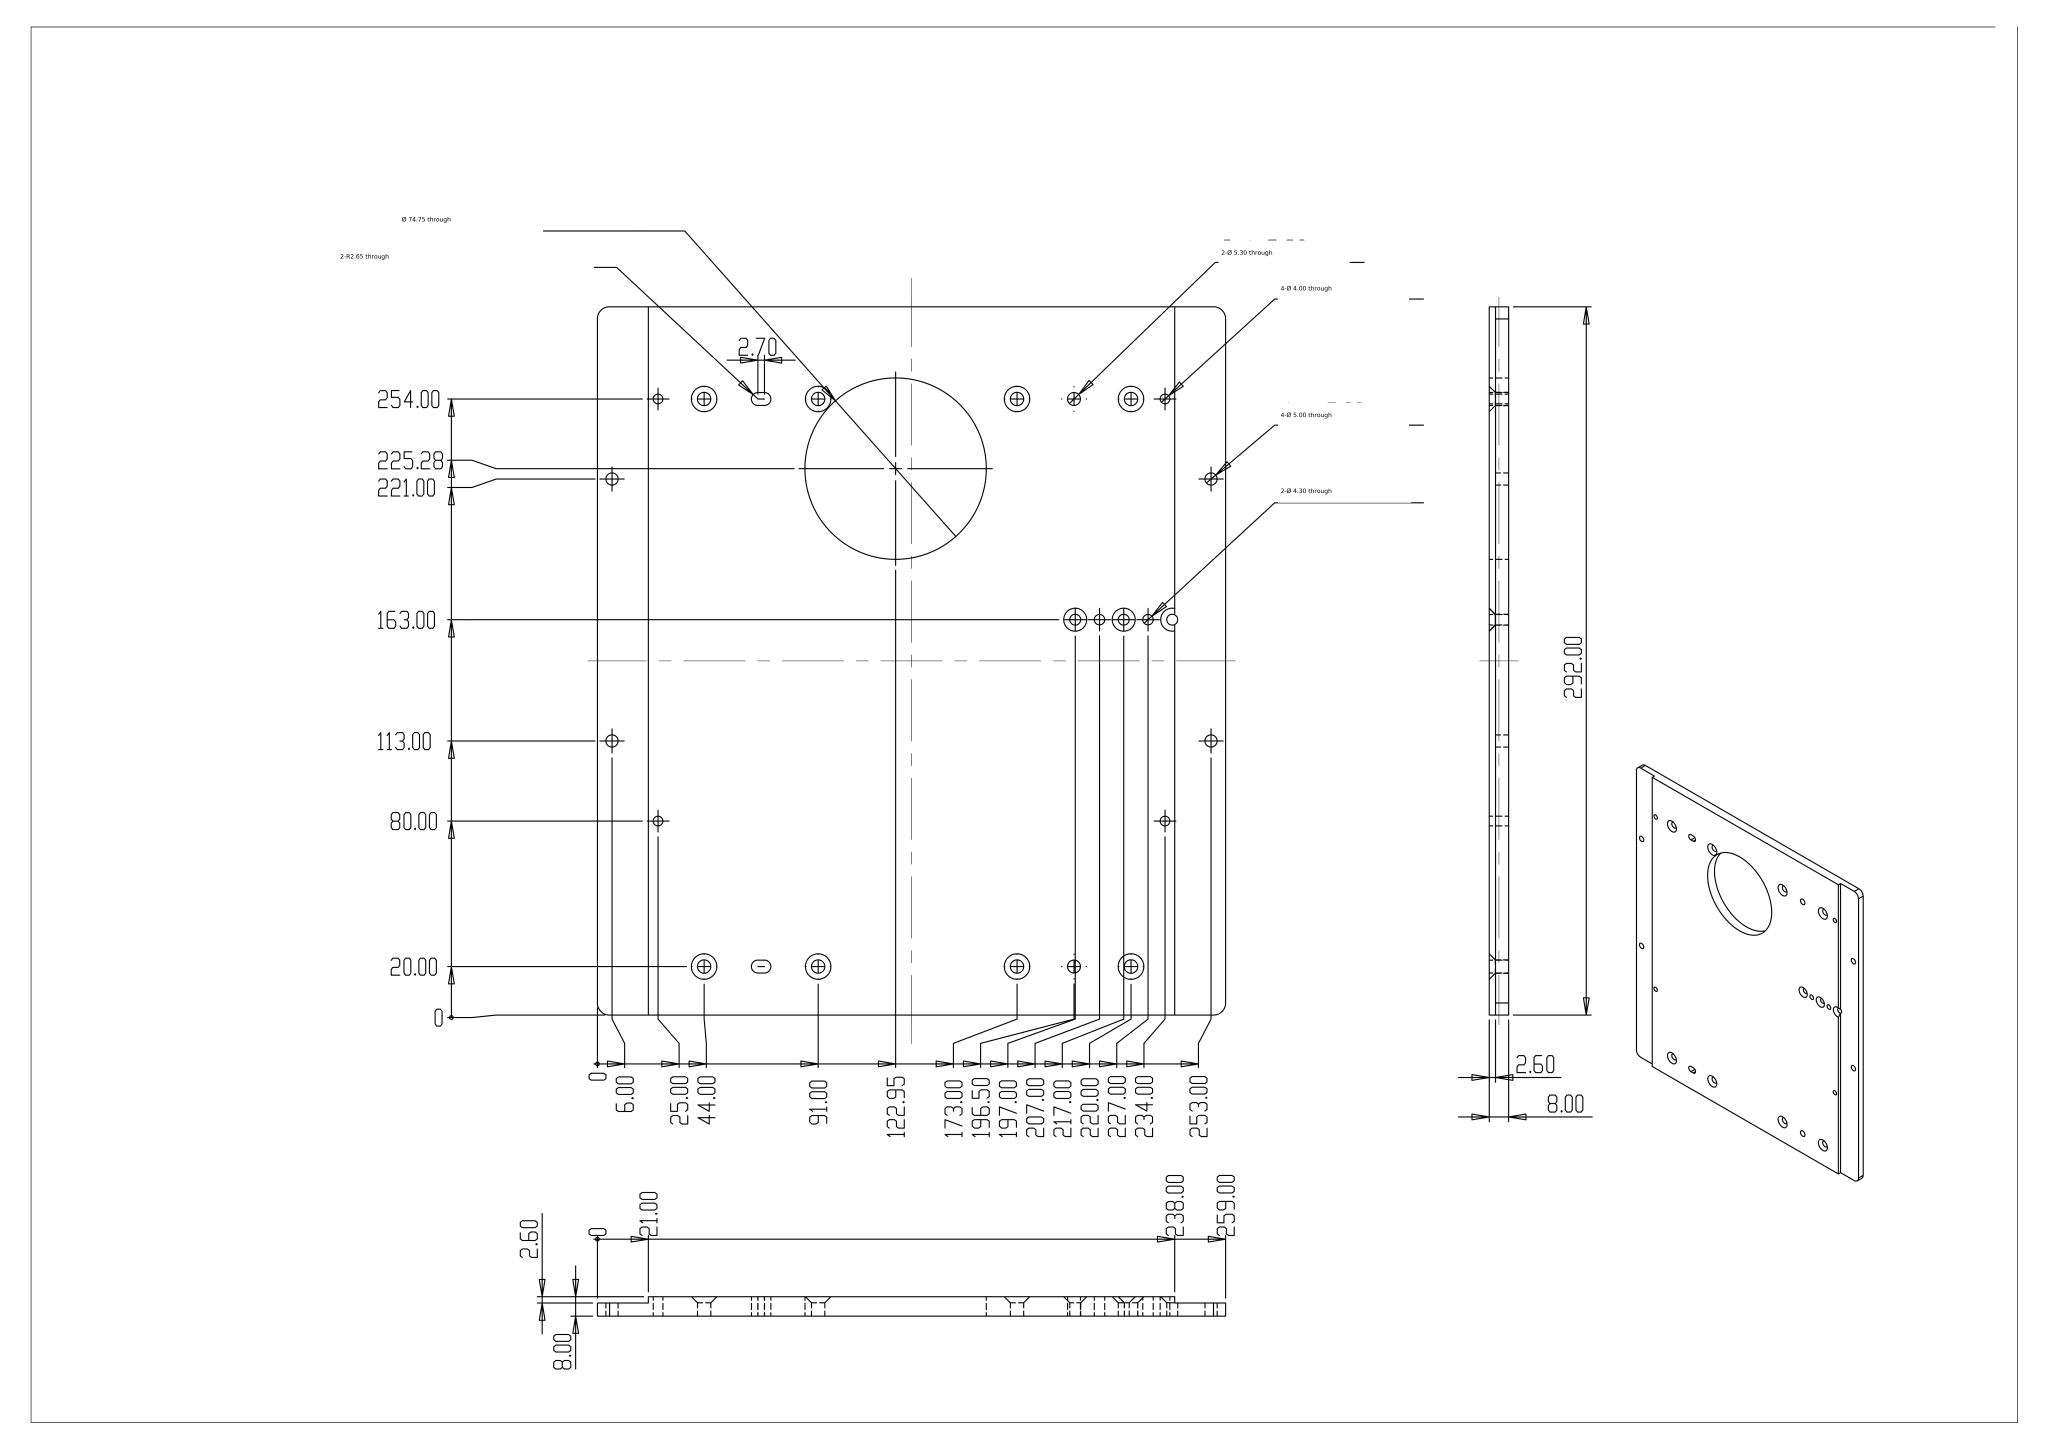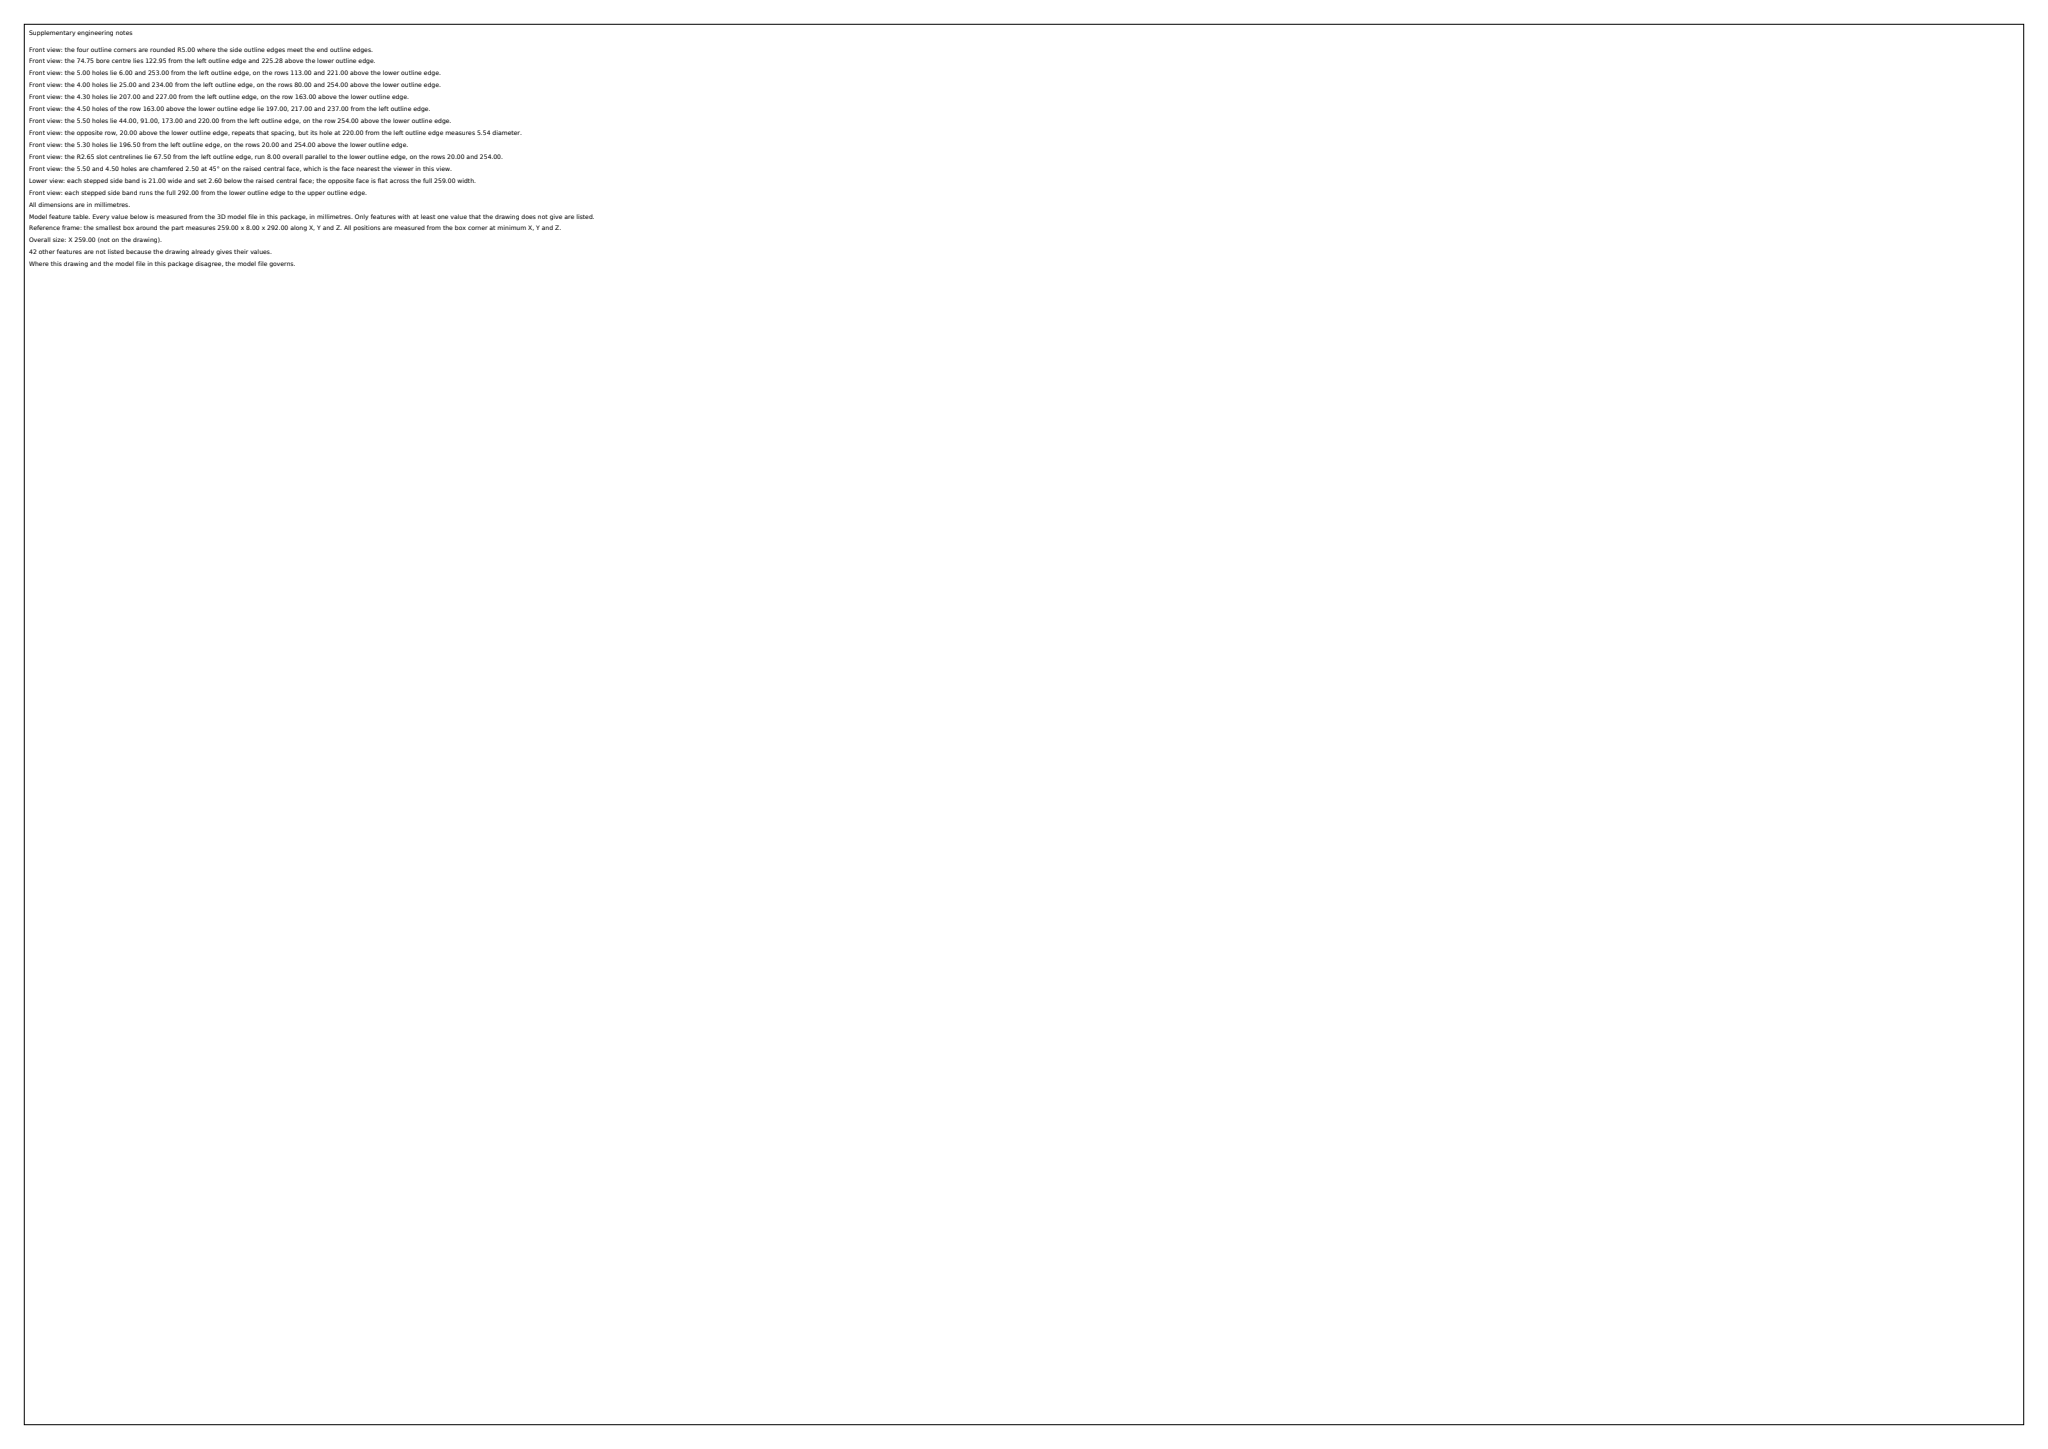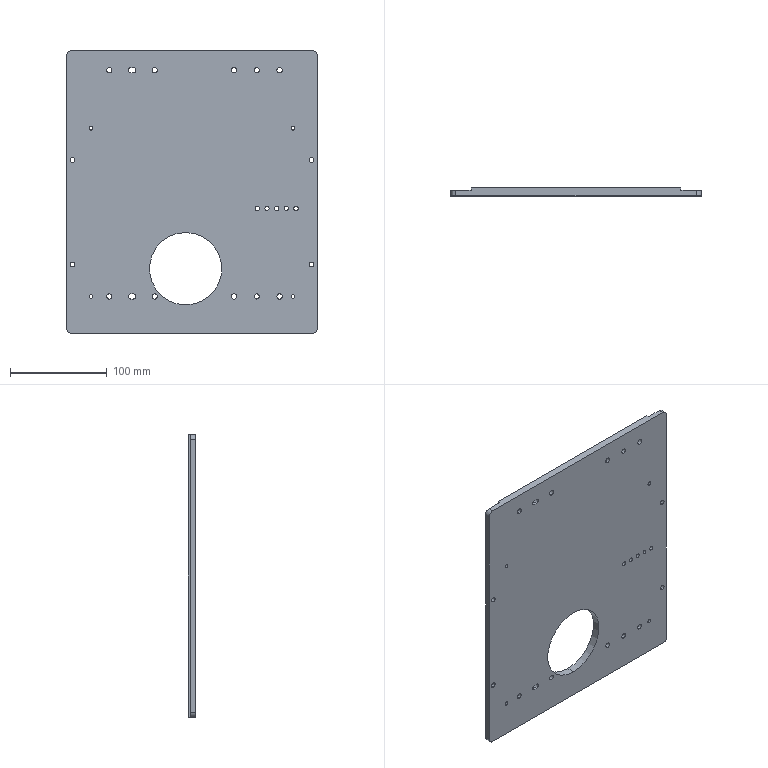Part | SolidWorks | mm | 1 solid | 94 faces | box 259 x 8 x 292 mm | volume 533304 mm3 | cylinder 56 | cone 23 | plane 15 | commonest cylinder face diameters 5.5 x14 4 x8 5.3 x8 5 x8 4.5 x6 4.3 x4 10 x4 74.75 x2
Drawing notes:
2X OBROUND SLOT 5.30 WIDE X 8.00 LONG (R2.65 ENDS, 2.70 BETWEEN ARC CENTRES), THRU; SLOT CENTRE AT X67.50 FROM LEFT EDGE DATUM; ONE SLOT ON TOP ROW Y254.00, ONE ON BOTTOM ROW Y20.00 | from the solid: cylinders dia 5.30 axis y at x=66.15 and x=68.85 (z=272 and z=38), length 8.00 (full plate thickness)
THIRD OF THE 3X Ø4.50 THRU, CSK Ø9.50 X 90° HOLES LOCATED AT X237.00 FROM LEFT EDGE DATUM, SAME ROW AS THE X197.00 AND X217.00 HOLES | from the solid: cylinder dia 4.50 axis y at x=237.0, z=129.0, length 5.5
ALL COUNTERSINKS (Ø10.50 X 90° ON THE Ø5.50 HOLES AND Ø9.50 X 90° ON THE Ø4.50 HOLES) ARE 2.50 DEEP AND APPLIED FROM ONE FACE ONLY, LEAVING A 5.50 LONG STRAIGHT HOLE IN THE 8.00 THICK PLATE | from the solid: cylinders dia 5.50 and 4.50 have length 5.5 while plate thickness (bbox y) = 8.001; cones 90° ref dia 5.5 and 4.5
build123d program:
from build123d import *

# Parameters (mm, degrees)
BOSS_EXTRUDE1_DEPTH = 292
SKETCH2_R           = 2.768
SKETCH2_R_2         = 2.75
SKETCH2_R_3         = 2
SKETCH2_R_4         = 2.25
CUT_EXTRUDE1_DEPTH  = 8
CHAMFER1_SIZE       = 2.5
CUT_EXTRUDE2_REACH  = 321.528
SKETCH3_R           = 37.375


with BuildPart() as part:
    # Sketch1 → Boss-Extrude1 (new body)
    with BuildSketch(Plane.XY):
        Polygon((129.5, 1.4), (124.5, 1.4), (108.5, 1.4), (108.5, 4), (-108.5, 4), (-108.5, 1.4), (-124.5, 1.4), (-129.5, 1.4), (-129.5, -4), (-124.5, -4), (124.5, -4), (129.5, -4), align=None)
    extrude(amount=BOSS_EXTRUDE1_DEPTH)

    # Sketch2 → Cut-Extrude1 (cut)
    with BuildSketch(Plane(origin=(0, 4, 0), x_dir=(1, 0, 0), z_dir=(0, 1, 0))):
        with Locations(Location((90.5, -272, 0), (0, 0, 270))):
            Circle(SKETCH2_R)
        with Locations(Location((43.5, -272, 0), (0, 0, 270))):
            Circle(SKETCH2_R_2)
        with Locations(Location((-38.5, -272, 0), (0, 0, 270))):
            Circle(SKETCH2_R_2)
        with Locations(Location((-85.5, -272, 0), (0, 0, 270))):
            Circle(SKETCH2_R_2)
        with Locations(Location((-104.5, -212, 0), (0, 0, 270))):
            Circle(SKETCH2_R_3)
        with Locations(Location((104.5, -212, 0), (0, 0, 270))):
            Circle(SKETCH2_R_3)
        with Locations(Location((67.5, -129, 0), (0, 0, 270))):
            Circle(SKETCH2_R_4)
        with Locations(Location((87.5, -129, 0), (0, 0, 270))):
            Circle(SKETCH2_R_4)
        with Locations(Location((107.5, -129, 0), (0, 0, 270))):
            Circle(SKETCH2_R_4)
        with Locations(Location((-104.5, -38, 0), (0, 0, 270))):
            Circle(SKETCH2_R_3)
        with Locations(Location((-85.5, -38, 0), (0, 0, 270))):
            Circle(SKETCH2_R_2)
        with Locations(Location((-38.5, -38, 0), (0, 0, 270))):
            Circle(SKETCH2_R_2)
        with Locations(Location((43.5, -38, 0), (0, 0, 270))):
            Circle(SKETCH2_R_2)
        with Locations(Location((90.5, -38, 0), (0, 0, 270))):
            Circle(SKETCH2_R_2)
        with Locations(Location((104.5, -38, 0), (0, 0, 270))):
            Circle(SKETCH2_R_3)
        with BuildLine():
            Line((-124.5, 0), (-129.5, 0))
            Line((-129.5, 0), (-129.5, -5))
            ThreePointArc((-129.5, -5), (-128.036, -1.464), (-124.5, 0))
        make_face()
        with BuildLine():
            Line((124.5, 0), (129.5, 0))
            Line((129.5, 0), (129.5, -5))
            ThreePointArc((129.5, -5), (128.036, -1.464), (124.5, 0))
        make_face()
        with BuildLine():
            Line((124.5, -292), (129.5, -292))
            Line((129.5, -292), (129.5, -287))
            ThreePointArc((129.5, -287), (128.036, -290.536), (124.5, -292))
        make_face()
        with BuildLine():
            Line((-129.5, -287), (-129.5, -292))
            Line((-129.5, -292), (-124.5, -292))
            ThreePointArc((-124.5, -292), (-128.036, -290.536), (-129.5, -287))
        make_face()
        with BuildLine():
            Line((-63.35, -274.65), (-60.65, -274.65))
            ThreePointArc((-60.65, -274.65), (-58, -272), (-60.65, -269.35))
            Line((-60.65, -269.35), (-63.35, -269.35))
            ThreePointArc((-63.35, -269.35), (-66, -272), (-63.35, -274.65))
        make_face()
        with BuildLine():
            Line((-63.35, -40.65), (-60.65, -40.65))
            ThreePointArc((-60.65, -40.65), (-58, -38), (-60.65, -35.35))
            Line((-60.65, -35.35), (-63.35, -35.35))
            ThreePointArc((-63.35, -35.35), (-66, -38), (-63.35, -40.65))
        make_face()
        with BuildLine():
            ThreePointArc((126, -179), (123.5, -176.5), (121, -179))
            ThreePointArc((121, -179), (123.5, -181.5), (126, -179))
        make_face()
        with BuildLine():
            ThreePointArc((126, -71), (123.5, -68.5), (121, -71))
            ThreePointArc((121, -71), (123.5, -73.5), (126, -71))
        make_face()
        with BuildLine():
            ThreePointArc((67, -274.65), (69.65, -272), (67, -269.35))
            ThreePointArc((67, -269.35), (64.35, -272), (67, -274.65))
        make_face()
        with BuildLine():
            ThreePointArc((77.5, -126.85), (75.35, -129), (77.5, -131.15))
            ThreePointArc((77.5, -131.15), (79.65, -129), (77.5, -126.85))
        make_face()
        with BuildLine():
            ThreePointArc((97.5, -126.85), (95.35, -129), (97.5, -131.15))
            ThreePointArc((97.5, -131.15), (99.65, -129), (97.5, -126.85))
        make_face()
        with BuildLine():
            ThreePointArc((67, -40.65), (69.65, -38), (67, -35.35))
            ThreePointArc((67, -35.35), (64.35, -38), (67, -40.65))
        make_face()
        with BuildLine():
            ThreePointArc((-121, -71), (-123.5, -68.5), (-126, -71))
            ThreePointArc((-126, -71), (-123.5, -73.5), (-121, -71))
        make_face()
        with BuildLine():
            ThreePointArc((-121, -179), (-123.5, -176.5), (-126, -179))
            ThreePointArc((-126, -179), (-123.5, -181.5), (-121, -179))
        make_face()
    extrude(amount=-CUT_EXTRUDE1_DEPTH, mode=Mode.SUBTRACT)

    # Chamfer1
    chamfer1_edges = [part.edges().sort_by_distance(p)[0] for p in [
        (67.5, 4, 126.75),
        (87.5, 4, 126.75),
        (105.309, 4, 128.486),
        (-85.5, 4, 269.25),
        (-38.5, 4, 269.25),
        (90.5, 4, 269.232),
        (43.5, 4, 269.25),
        (90.5, 4, 35.25),
        (43.5, 4, 35.25),
        (-38.5, 4, 35.25),
        (-85.5, 4, 35.25),
    ]]
    chamfer(chamfer1_edges, length=CHAMFER1_SIZE)

    # Sketch3 → Cut-Extrude2 (cut, up to next)
    with BuildSketch(Plane(origin=(0, 4, 0), x_dir=(1, 0, 0), z_dir=(0, 1, 0)), mode=Mode.PRIVATE) as cut_extrude2_sk1:
        with Locations(Location((-6.55, -66.72, 0), (0, 0, 270))):
            Circle(SKETCH3_R)
    cut_extrude2_tool1 = extrude(cut_extrude2_sk1.sketch, amount=-CUT_EXTRUDE2_REACH, mode=Mode.PRIVATE) & part.part
    add(cut_extrude2_tool1.solids().sort_by_distance((-6.55, 4, 66.72))[0], mode=Mode.SUBTRACT)


solid = part.part